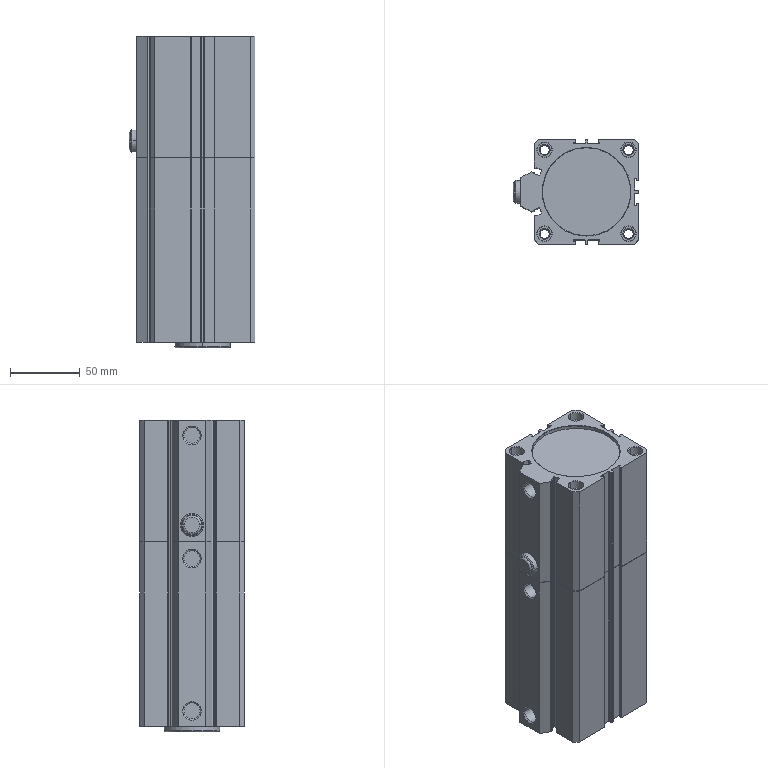Component | SolidWorks | NewCurveBenderSDAT63x45x45Cylinder-DoubleWheel-1_NewTypeCurveBenderSDATS-63x45x45_4545b-DoubleWheel-1 | 1 solid | 505 faces | box 90.1 x 75 x 223 mm | volume 609887 mm3 | plane 212 | cylinder 211 | cone 78 | torus 4 | commonest cylinder face diameters 0.4 x106 10.5 x32 0.8 x17 6.647 x16 11.445 x8 8 x8 6.5 x8 63 x6
build123d program:
from build123d import *

# Parameters (mm, degrees)
BOSS_EXTRUDE1_DEPTH     = 219
CUT_EXTRUDE1_DEPTH      = 0.1
CUT_EXTRUDE1_DEPTH_BACK = 0.1
SKETCH2_W               = 120
SKETCH2_H               = 120
LPATTERN1_COUNT         = 2
LPATTERN1_PITCH         = 60
LPATTERN1_COUNT_DIR2    = 2
LPATTERN1_PITCH_DIR2    = 60
LPATTERN2_COUNT         = 2
LPATTERN2_PITCH         = 60
LPATTERN2_COUNT_DIR2    = 2
LPATTERN2_PITCH_DIR2    = 60
LPATTERN3_COUNT         = 2
LPATTERN3_PITCH         = 60
LPATTERN3_COUNT_DIR2    = 2
LPATTERN3_PITCH_DIR2    = 60
HOLE1_D                 = 11.445
HOLE1_DEPTH             = 8
HOLE1_CSINK_D           = 13.157
HOLE1_CSINK_ANGLE       = 90
HOLE2_D                 = 11.445
HOLE2_DEPTH             = 8
HOLE2_CSINK_D           = 13.157
HOLE2_CSINK_ANGLE       = 90


with BuildPart() as part:
    # Sketch1 → Boss-Extrude1 (new body)
    with BuildSketch(Plane(origin=(0, 0, 0), x_dir=(0, 0, -1), z_dir=(1, 0, 0))):
        with BuildLine():
            Line((-37.5, 0.8), (-37.5, -0.8))
            ThreePointArc((-37.5, -0.8), (-37.441, -0.9414), (-37.3, -1))
            Line((-37.3, -1), (-34.7, -1))
            ThreePointArc((-34.7, -1), (-34.559, -1.059), (-34.5, -1.2))
            Line((-34.5, -1.2), (-34.5, -9.4))
            ThreePointArc((-34.5, -9.4), (-34.559, -9.541), (-34.7, -9.6))
            Line((-34.7, -9.6), (-35.3, -9.6))
            ThreePointArc((-35.3, -9.6), (-35.441, -9.541), (-35.5, -9.4))
            Line((-35.5, -9.4), (-35.5, -8.4))
            ThreePointArc((-35.5, -8.4), (-35.559, -8.259), (-35.7, -8.2))
            Line((-35.7, -8.2), (-37.3, -8.2))
            ThreePointArc((-37.3, -8.2), (-37.441, -8.259), (-37.5, -8.4))
            Line((-37.5, -8.4), (-37.5, -34.3))
            Line((-37.5, -34.3), (-34.3, -37.5))
            Line((-34.3, -37.5), (-8.4, -37.5))
            ThreePointArc((-8.4, -37.5), (-8.259, -37.441), (-8.2, -37.3))
            Line((-8.2, -37.3), (-8.2, -35.7))
            ThreePointArc((-8.2, -35.7), (-8.259, -35.559), (-8.4, -35.5))
            Line((-8.4, -35.5), (-9.4, -35.5))
            ThreePointArc((-9.4, -35.5), (-9.541, -35.441), (-9.6, -35.3))
            Line((-9.6, -35.3), (-9.6, -34.7))
            ThreePointArc((-9.6, -34.7), (-9.541, -34.559), (-9.4, -34.5))
            Line((-9.4, -34.5), (-1.2, -34.5))
            ThreePointArc((-1.2, -34.5), (-1.059, -34.559), (-1, -34.7))
            Line((-1, -34.7), (-1, -37.3))
            ThreePointArc((-1, -37.3), (-0.9414, -37.441), (-0.8, -37.5))
            Line((-0.8, -37.5), (0.8, -37.5))
            ThreePointArc((0.8, -37.5), (0.9414, -37.441), (1, -37.3))
            Line((1, -37.3), (1, -34.7))
            ThreePointArc((1, -34.7), (1.059, -34.559), (1.2, -34.5))
            Line((1.2, -34.5), (9.4, -34.5))
            ThreePointArc((9.4, -34.5), (9.541, -34.559), (9.6, -34.7))
            Line((9.6, -34.7), (9.6, -35.3))
            ThreePointArc((9.6, -35.3), (9.541, -35.441), (9.4, -35.5))
            Line((9.4, -35.5), (8.4, -35.5))
            ThreePointArc((8.4, -35.5), (8.259, -35.559), (8.2, -35.7))
            Line((8.2, -35.7), (8.2, -37.3))
            ThreePointArc((8.2, -37.3), (8.259, -37.441), (8.4, -37.5))
            Line((8.4, -37.5), (34.3, -37.5))
            Line((34.3, -37.5), (37.5, -34.3))
            Line((37.5, -34.3), (37.5, -8.4))
            ThreePointArc((37.5, -8.4), (37.441, -8.259), (37.3, -8.2))
            Line((37.3, -8.2), (35.7, -8.2))
            ThreePointArc((35.7, -8.2), (35.559, -8.259), (35.5, -8.4))
            Line((35.5, -8.4), (35.5, -9.4))
            ThreePointArc((35.5, -9.4), (35.441, -9.541), (35.3, -9.6))
            Line((35.3, -9.6), (34.7, -9.6))
            ThreePointArc((34.7, -9.6), (34.559, -9.541), (34.5, -9.4))
            Line((34.5, -9.4), (34.5, -1.2))
            ThreePointArc((34.5, -1.2), (34.559, -1.059), (34.7, -1))
            Line((34.7, -1), (37.3, -1))
            ThreePointArc((37.3, -1), (37.441, -0.9414), (37.5, -0.8))
            Line((37.5, -0.8), (37.5, 0.8))
            ThreePointArc((37.5, 0.8), (37.441, 0.9414), (37.3, 1))
            Line((37.3, 1), (34.7, 1))
            ThreePointArc((34.7, 1), (34.559, 1.059), (34.5, 1.2))
            Line((34.5, 1.2), (34.5, 9.4))
            ThreePointArc((34.5, 9.4), (34.559, 9.541), (34.7, 9.6))
            Line((34.7, 9.6), (35.3, 9.6))
            ThreePointArc((35.3, 9.6), (35.441, 9.541), (35.5, 9.4))
            Line((35.5, 9.4), (35.5, 8.4))
            ThreePointArc((35.5, 8.4), (35.559, 8.259), (35.7, 8.2))
            Line((35.7, 8.2), (37.3, 8.2))
            ThreePointArc((37.3, 8.2), (37.441, 8.259), (37.5, 8.4))
            Line((37.5, 8.4), (37.5, 34.3))
            Line((37.5, 34.3), (34.3, 37.5))
            Line((34.3, 37.5), (17.64, 37.5))
            ThreePointArc((17.64, 37.5), (17.418, 37.433), (17.271, 37.253))
            Line((17.271, 37.253), (16.878, 36.305))
            ThreePointArc((16.878, 36.305), (16.878, 36.152), (16.986, 36.043))
            Line((16.986, 36.043), (17.171, 35.967))
            ThreePointArc((17.171, 35.967), (17.279, 35.859), (17.279, 35.705))
            Line((17.279, 35.705), (15.863, 32.287))
            ThreePointArc((15.863, 32.287), (15.647, 32.071), (15.341, 32.071))
            Line((15.341, 32.071), (11.83, 33.525))
            ThreePointArc((11.83, 33.525), (11.613, 33.741), (11.613, 34.047))
            Line((11.613, 34.047), (13.029, 37.466))
            ThreePointArc((13.029, 37.466), (13.138, 37.574), (13.291, 37.574))
            Line((13.291, 37.574), (13.46, 37.504))
            ThreePointArc((13.46, 37.504), (13.62, 37.507), (13.727, 37.627))
            Line((13.727, 37.627), (14.276, 39.331))
            ThreePointArc((14.276, 39.331), (14.293, 39.496), (14.241, 39.654))
            Line((14.241, 39.654), (10, 47))
            Line((10, 47), (-10, 47))
            Line((-10, 47), (-14.241, 39.654))
            ThreePointArc((-14.241, 39.654), (-14.293, 39.496), (-14.276, 39.331))
            Line((-14.276, 39.331), (-13.727, 37.627))
            ThreePointArc((-13.727, 37.627), (-13.62, 37.507), (-13.46, 37.504))
            Line((-13.46, 37.504), (-13.291, 37.574))
            ThreePointArc((-13.291, 37.574), (-13.138, 37.574), (-13.029, 37.466))
            Line((-13.029, 37.466), (-11.613, 34.047))
            ThreePointArc((-11.613, 34.047), (-11.613, 33.741), (-11.83, 33.525))
            Line((-11.83, 33.525), (-15.341, 32.071))
            ThreePointArc((-15.341, 32.071), (-15.647, 32.071), (-15.863, 32.287))
            Line((-15.863, 32.287), (-17.279, 35.705))
            ThreePointArc((-17.279, 35.705), (-17.279, 35.859), (-17.171, 35.967))
            Line((-17.171, 35.967), (-16.986, 36.043))
            ThreePointArc((-16.986, 36.043), (-16.878, 36.152), (-16.878, 36.305))
            Line((-16.878, 36.305), (-17.271, 37.253))
            ThreePointArc((-17.271, 37.253), (-17.418, 37.433), (-17.64, 37.5))
            Line((-17.64, 37.5), (-34.3, 37.5))
            Line((-34.3, 37.5), (-37.5, 34.3))
            Line((-37.5, 34.3), (-37.5, 8.4))
            ThreePointArc((-37.5, 8.4), (-37.441, 8.259), (-37.3, 8.2))
            Line((-37.3, 8.2), (-35.7, 8.2))
            ThreePointArc((-35.7, 8.2), (-35.559, 8.259), (-35.5, 8.4))
            Line((-35.5, 8.4), (-35.5, 9.4))
            ThreePointArc((-35.5, 9.4), (-35.441, 9.541), (-35.3, 9.6))
            Line((-35.3, 9.6), (-34.7, 9.6))
            ThreePointArc((-34.7, 9.6), (-34.559, 9.541), (-34.5, 9.4))
            Line((-34.5, 9.4), (-34.5, 1.2))
            ThreePointArc((-34.5, 1.2), (-34.559, 1.059), (-34.7, 1))
            Line((-34.7, 1), (-37.3, 1))
            ThreePointArc((-37.3, 1), (-37.441, 0.9414), (-37.5, 0.8))
        make_face()
    extrude(amount=BOSS_EXTRUDE1_DEPTH)

    # Sketch2 → Cut-Extrude1 (cut, two sides: drawn at the far end of the back side and taken through both)
    with BuildSketch(Plane(origin=(132, 0, 0), x_dir=(0, 0, -1), z_dir=(1, 0, 0)).offset(-CUT_EXTRUDE1_DEPTH_BACK)):
        Rectangle(SKETCH2_W, SKETCH2_H)
        with BuildLine():
            Line((-37.3, 0.6), (-37.3, -0.6))
            ThreePointArc((-37.3, -0.6), (-37.241, -0.7414), (-37.1, -0.8))
            Line((-37.1, -0.8), (-34.5, -0.8))
            ThreePointArc((-34.5, -0.8), (-34.359, -0.8586), (-34.3, -1))
            Line((-34.3, -1), (-34.3, -9.8))
            ThreePointArc((-34.3, -9.8), (-34.359, -9.941), (-34.5, -10))
            Line((-34.5, -10), (-35.1, -10))
            ThreePointArc((-35.1, -10), (-35.241, -9.941), (-35.3, -9.8))
            Line((-35.3, -9.8), (-35.3, -8.8))
            ThreePointArc((-35.3, -8.8), (-35.359, -8.659), (-35.5, -8.6))
            Line((-35.5, -8.6), (-37.1, -8.6))
            ThreePointArc((-37.1, -8.6), (-37.241, -8.659), (-37.3, -8.8))
            Line((-37.3, -8.8), (-37.3, -34.1))
            Line((-37.3, -34.1), (-34.1, -37.3))
            Line((-34.1, -37.3), (-8.8, -37.3))
            ThreePointArc((-8.8, -37.3), (-8.659, -37.241), (-8.6, -37.1))
            Line((-8.6, -37.1), (-8.6, -35.5))
            ThreePointArc((-8.6, -35.5), (-8.659, -35.359), (-8.8, -35.3))
            Line((-8.8, -35.3), (-9.8, -35.3))
            ThreePointArc((-9.8, -35.3), (-9.941, -35.241), (-10, -35.1))
            Line((-10, -35.1), (-10, -34.5))
            ThreePointArc((-10, -34.5), (-9.941, -34.359), (-9.8, -34.3))
            Line((-9.8, -34.3), (-1, -34.3))
            ThreePointArc((-1, -34.3), (-0.8586, -34.359), (-0.8, -34.5))
            Line((-0.8, -34.5), (-0.8, -37.1))
            ThreePointArc((-0.8, -37.1), (-0.7414, -37.241), (-0.6, -37.3))
            Line((-0.6, -37.3), (0.6, -37.3))
            ThreePointArc((0.6, -37.3), (0.7414, -37.241), (0.8, -37.1))
            Line((0.8, -37.1), (0.8, -34.5))
            ThreePointArc((0.8, -34.5), (0.8586, -34.359), (1, -34.3))
            Line((1, -34.3), (9.8, -34.3))
            ThreePointArc((9.8, -34.3), (9.941, -34.359), (10, -34.5))
            Line((10, -34.5), (10, -35.1))
            ThreePointArc((10, -35.1), (9.941, -35.241), (9.8, -35.3))
            Line((9.8, -35.3), (8.8, -35.3))
            ThreePointArc((8.8, -35.3), (8.659, -35.359), (8.6, -35.5))
            Line((8.6, -35.5), (8.6, -37.1))
            ThreePointArc((8.6, -37.1), (8.659, -37.241), (8.8, -37.3))
            Line((8.8, -37.3), (34.1, -37.3))
            Line((34.1, -37.3), (37.3, -34.1))
            Line((37.3, -34.1), (37.3, -8.8))
            ThreePointArc((37.3, -8.8), (37.241, -8.659), (37.1, -8.6))
            Line((37.1, -8.6), (35.5, -8.6))
            ThreePointArc((35.5, -8.6), (35.359, -8.659), (35.3, -8.8))
            Line((35.3, -8.8), (35.3, -9.8))
            ThreePointArc((35.3, -9.8), (35.241, -9.941), (35.1, -10))
            Line((35.1, -10), (34.5, -10))
            ThreePointArc((34.5, -10), (34.359, -9.941), (34.3, -9.8))
            Line((34.3, -9.8), (34.3, -1))
            ThreePointArc((34.3, -1), (34.359, -0.8586), (34.5, -0.8))
            Line((34.5, -0.8), (37.1, -0.8))
            ThreePointArc((37.1, -0.8), (37.241, -0.7414), (37.3, -0.6))
            Line((37.3, -0.6), (37.3, 0.6))
            ThreePointArc((37.3, 0.6), (37.241, 0.7414), (37.1, 0.8))
            Line((37.1, 0.8), (34.5, 0.8))
            ThreePointArc((34.5, 0.8), (34.359, 0.8586), (34.3, 1))
            Line((34.3, 1), (34.3, 9.8))
            ThreePointArc((34.3, 9.8), (34.359, 9.941), (34.5, 10))
            Line((34.5, 10), (35.1, 10))
            ThreePointArc((35.1, 10), (35.241, 9.941), (35.3, 9.8))
            Line((35.3, 9.8), (35.3, 8.8))
            ThreePointArc((35.3, 8.8), (35.359, 8.659), (35.5, 8.6))
            Line((35.5, 8.6), (37.1, 8.6))
            ThreePointArc((37.1, 8.6), (37.241, 8.659), (37.3, 8.8))
            Line((37.3, 8.8), (37.3, 34.1))
            Line((37.3, 34.1), (34.1, 37.3))
            Line((34.1, 37.3), (17.558, 37.3))
            ThreePointArc((17.558, 37.3), (17.335, 37.233), (17.188, 37.053))
            Line((17.188, 37.053), (16.878, 36.305))
            ThreePointArc((16.878, 36.305), (16.878, 36.152), (16.986, 36.043))
            Line((16.986, 36.043), (17.171, 35.967))
            ThreePointArc((17.171, 35.967), (17.279, 35.859), (17.279, 35.705))
            Line((17.279, 35.705), (15.863, 32.287))
            ThreePointArc((15.863, 32.287), (15.647, 32.071), (15.341, 32.071))
            Line((15.341, 32.071), (11.83, 33.525))
            ThreePointArc((11.83, 33.525), (11.613, 33.741), (11.613, 34.047))
            Line((11.613, 34.047), (13.029, 37.466))
            ThreePointArc((13.029, 37.466), (13.138, 37.574), (13.291, 37.574))
            Line((13.291, 37.574), (13.466, 37.501))
            ThreePointArc((13.466, 37.501), (13.624, 37.503), (13.731, 37.619))
            Line((13.731, 37.619), (14.268, 39.126))
            ThreePointArc((14.268, 39.126), (14.29, 39.296), (14.238, 39.46))
            Line((14.238, 39.46), (10, 46.8))
            Line((10, 46.8), (-10, 46.8))
            Line((-10, 46.8), (-14.238, 39.46))
            ThreePointArc((-14.238, 39.46), (-14.29, 39.296), (-14.268, 39.126))
            Line((-14.268, 39.126), (-13.731, 37.619))
            ThreePointArc((-13.731, 37.619), (-13.624, 37.503), (-13.466, 37.501))
            Line((-13.466, 37.501), (-13.291, 37.574))
            ThreePointArc((-13.291, 37.574), (-13.138, 37.574), (-13.029, 37.466))
            Line((-13.029, 37.466), (-11.613, 34.047))
            ThreePointArc((-11.613, 34.047), (-11.613, 33.741), (-11.83, 33.525))
            Line((-11.83, 33.525), (-15.341, 32.071))
            ThreePointArc((-15.341, 32.071), (-15.647, 32.071), (-15.863, 32.287))
            Line((-15.863, 32.287), (-17.279, 35.705))
            ThreePointArc((-17.279, 35.705), (-17.279, 35.859), (-17.171, 35.967))
            Line((-17.171, 35.967), (-16.986, 36.043))
            ThreePointArc((-16.986, 36.043), (-16.878, 36.152), (-16.878, 36.305))
            Line((-16.878, 36.305), (-17.188, 37.053))
            ThreePointArc((-17.188, 37.053), (-17.335, 37.233), (-17.558, 37.3))
            Line((-17.558, 37.3), (-34.1, 37.3))
            Line((-34.1, 37.3), (-37.3, 34.1))
            Line((-37.3, 34.1), (-37.3, 8.8))
            ThreePointArc((-37.3, 8.8), (-37.241, 8.659), (-37.1, 8.6))
            Line((-37.1, 8.6), (-35.5, 8.6))
            ThreePointArc((-35.5, 8.6), (-35.359, 8.659), (-35.3, 8.8))
            Line((-35.3, 8.8), (-35.3, 9.8))
            ThreePointArc((-35.3, 9.8), (-35.241, 9.941), (-35.1, 10))
            Line((-35.1, 10), (-34.5, 10))
            ThreePointArc((-34.5, 10), (-34.359, 9.941), (-34.3, 9.8))
            Line((-34.3, 9.8), (-34.3, 1))
            ThreePointArc((-34.3, 1), (-34.359, 0.8586), (-34.5, 0.8))
            Line((-34.5, 0.8), (-37.1, 0.8))
            ThreePointArc((-37.1, 0.8), (-37.241, 0.7414), (-37.3, 0.6))
        make_face(mode=Mode.SUBTRACT)
    extrude(amount=CUT_EXTRUDE1_DEPTH + CUT_EXTRUDE1_DEPTH_BACK, mode=Mode.SUBTRACT)

    # Sketch3 → Cut-Revolve1 (revolve, cut)
    with BuildSketch(Plane.XY.offset(30), mode=Mode.PRIVATE) as cut_revolve1_sk:
        Polygon((0, -30), (0, -24.45), (0.3, -24.75), (6.5, -24.75), (6.5, -26), (7.176, -26.677), (24.323, -26.677), (25, -26), (25, -26.75), (66, -26.75), (66, -30), align=None)
    cut_revolve1 = revolve(cut_revolve1_sk.sketch.rotate(Axis((66, -30, 30), (-1, 0, 0)), 270), axis=Axis((66, -30, 30), (-1, 0, 0)), mode=Mode.SUBTRACT)

    # LPattern1: Cut-Revolve1 2 × 2
    with Locations(*[(0, j * LPATTERN1_PITCH_DIR2, -i * LPATTERN1_PITCH) for i in range(LPATTERN1_COUNT) for j in range(LPATTERN1_COUNT_DIR2) if (i, j) != (0, 0)]):
        add(cut_revolve1, mode=Mode.SUBTRACT)

    # Sketch5 → Cut-Revolve2 (revolve, cut)
    with BuildSketch(Plane.XY.offset(30), mode=Mode.PRIVATE) as cut_revolve2_sk:
        Polygon((66, -30), (66, -26.75), (107, -26.75), (107, -26), (107.677, -26.677), (124.823, -26.677), (125.5, -26), (125.5, -24.75), (131.7, -24.75), (132, -24.45), (132, -30), align=None)
    cut_revolve2 = revolve(cut_revolve2_sk.sketch.rotate(Axis((132, -30, 30), (-1, 0, 0)), 270), axis=Axis((132, -30, 30), (-1, 0, 0)), mode=Mode.SUBTRACT)

    # LPattern2: Cut-Revolve2 2 × 2
    with Locations(*[(0, j * LPATTERN2_PITCH_DIR2, -i * LPATTERN2_PITCH) for i in range(LPATTERN2_COUNT) for j in range(LPATTERN2_COUNT_DIR2) if (i, j) != (0, 0)]):
        add(cut_revolve2, mode=Mode.SUBTRACT)

    # Sketch7 → Cut-Revolve3 (revolve, cut)
    with BuildSketch(Plane.XY.offset(30), mode=Mode.PRIVATE) as cut_revolve3_sk:
        Polygon((132, -30), (132, -24.5), (132.25, -24.75), (138.5, -24.75), (138.5, -26), (212.5, -26), (212.5, -24.75), (218.75, -24.75), (219, -24.5), (219, -30), align=None)
    cut_revolve3 = revolve(cut_revolve3_sk.sketch.rotate(Axis((219, -30, 30), (-1, 0, 0)), 270), axis=Axis((219, -30, 30), (-1, 0, 0)), mode=Mode.SUBTRACT)

    # LPattern3: Cut-Revolve3 2 × 2
    with Locations(*[(0, j * LPATTERN3_PITCH_DIR2, -i * LPATTERN3_PITCH) for i in range(LPATTERN3_COUNT) for j in range(LPATTERN3_COUNT_DIR2) if (i, j) != (0, 0)]):
        add(cut_revolve3, mode=Mode.SUBTRACT)

    # Sketch9 → Cut-Revolve4 (revolve, cut)
    with BuildSketch(Plane.XY, mode=Mode.PRIVATE) as cut_revolve4_sk:
        Polygon((11, 47), (17.578, 47), (16.723, 46.144), (16.723, 39), (11, 39), align=None)
    revolve(cut_revolve4_sk.sketch.rotate(Axis((11, 39, 0), (0, 1, 0)), 270), axis=Axis((11, 39, 0), (0, 1, 0)), mode=Mode.SUBTRACT)

    # Hole1
    with Locations(Plane(origin=(0, 47, 0), x_dir=(1, 0, 0), z_dir=(0, 1, 0))):
        with Locations((120, 0)):
            CounterSinkHole(HOLE1_D / 2, HOLE1_CSINK_D / 2, depth=HOLE1_DEPTH, counter_sink_angle=HOLE1_CSINK_ANGLE)

    # Hole2
    with Locations(Plane(origin=(0, 47, 0), x_dir=(1, 0, 0), z_dir=(0, 1, 0))):
        with Locations((144, 0)):
            CounterSinkHole(HOLE2_D / 2, HOLE2_CSINK_D / 2, depth=HOLE2_DEPTH, counter_sink_angle=HOLE2_CSINK_ANGLE)

    # Sketch15 → Cut-Revolve5 (revolve, cut)
    with BuildSketch(Plane.XY, mode=Mode.PRIVATE) as cut_revolve5_sk:
        Polygon((208, 47), (214.578, 47), (213.722, 46.144), (213.722, 39), (208, 39), align=None)
    revolve(cut_revolve5_sk.sketch.rotate(Axis((208, 39, 0), (0, 1, 0)), 270), axis=Axis((208, 39, 0), (0, 1, 0)), mode=Mode.SUBTRACT)

    # Sketch16 → Revolve1 (revolve)
    with BuildSketch(Plane.XY, mode=Mode.PRIVATE) as revolve1_sk:
        with BuildLine():
            Line((144, 52.6), (149.5, 52.6))
            ThreePointArc((149.5, 52.6), (150.419, 52.219), (150.8, 51.3))
            Line((150.8, 51.3), (151.5, 51.3))
            Line((151.5, 51.3), (152.25, 50.55))
            Line((152.25, 50.55), (152.25, 47))
            Line((152.25, 47), (144, 47))
            Line((144, 47), (144, 52.6))
        make_face()
    revolve(revolve1_sk.sketch.rotate(Axis((144, 47, 0), (0, 1, 0)), 270), axis=Axis((144, 47, 0), (0, 1, 0)))

    # Sketch17 → Cut-Revolve6 (revolve, cut)
    with BuildSketch(Plane.XY, mode=Mode.PRIVATE) as cut_revolve6_sk:
        Polygon((0, 0), (0, 10), (9, 10), (9, 31.5), (122, 31.5), (122, 10), (141, 10), (141, 31.5), (209, 31.5), (209, 0), align=None)
    revolve(cut_revolve6_sk.sketch.rotate(Axis((209, 0, 0), (-1, 0, 0)), 270), axis=Axis((209, 0, 0), (-1, 0, 0)), mode=Mode.SUBTRACT)

    # Sketch18 → Cut-Revolve7 (revolve, cut)
    with BuildSketch(Plane.XY, mode=Mode.PRIVATE) as cut_revolve7_sk:
        Polygon((0, 0), (0, 33), (0.5, 32.5), (5, 32.5), (5, 0), align=None)
    revolve(cut_revolve7_sk.sketch.rotate(Axis((5, 0, 0), (-1, 0, 0)), 270), axis=Axis((5, 0, 0), (-1, 0, 0)), mode=Mode.SUBTRACT)

    # Sketch19 → Revolve2 (revolve)
    with BuildSketch(Plane.XY, mode=Mode.PRIVATE) as revolve2_sk:
        with BuildLine():
            Line((-4, 10), (5, 10))
            Line((5, 10), (5, 20))
            Line((5, 20), (-3, 20))
            ThreePointArc((-3, 20), (-3.707, 19.707), (-4, 19))
            Line((-4, 19), (-4, 10))
        make_face()
    revolve(revolve2_sk.sketch.rotate(Axis((5, 0, 0), (-1, 0, 0)), 270), axis=Axis((5, 0, 0), (-1, 0, 0)))

    # Sketch20 → Cut-Revolve8 (revolve, cut)
    with BuildSketch(Plane.XY, mode=Mode.PRIVATE) as cut_revolve8_sk:
        Polygon((216.5, 0), (216.5, 31.5), (218.75, 31.5), (219, 31.75), (219, 0), align=None)
    revolve(cut_revolve8_sk.sketch.rotate(Axis((219, 0, 0), (-1, 0, 0)), 270), axis=Axis((219, 0, 0), (-1, 0, 0)), mode=Mode.SUBTRACT)


solid = part.part

# Placed as in the assembly
solid = solid.moved(Location((0, 47, 281.11), (90, 0, 90)))